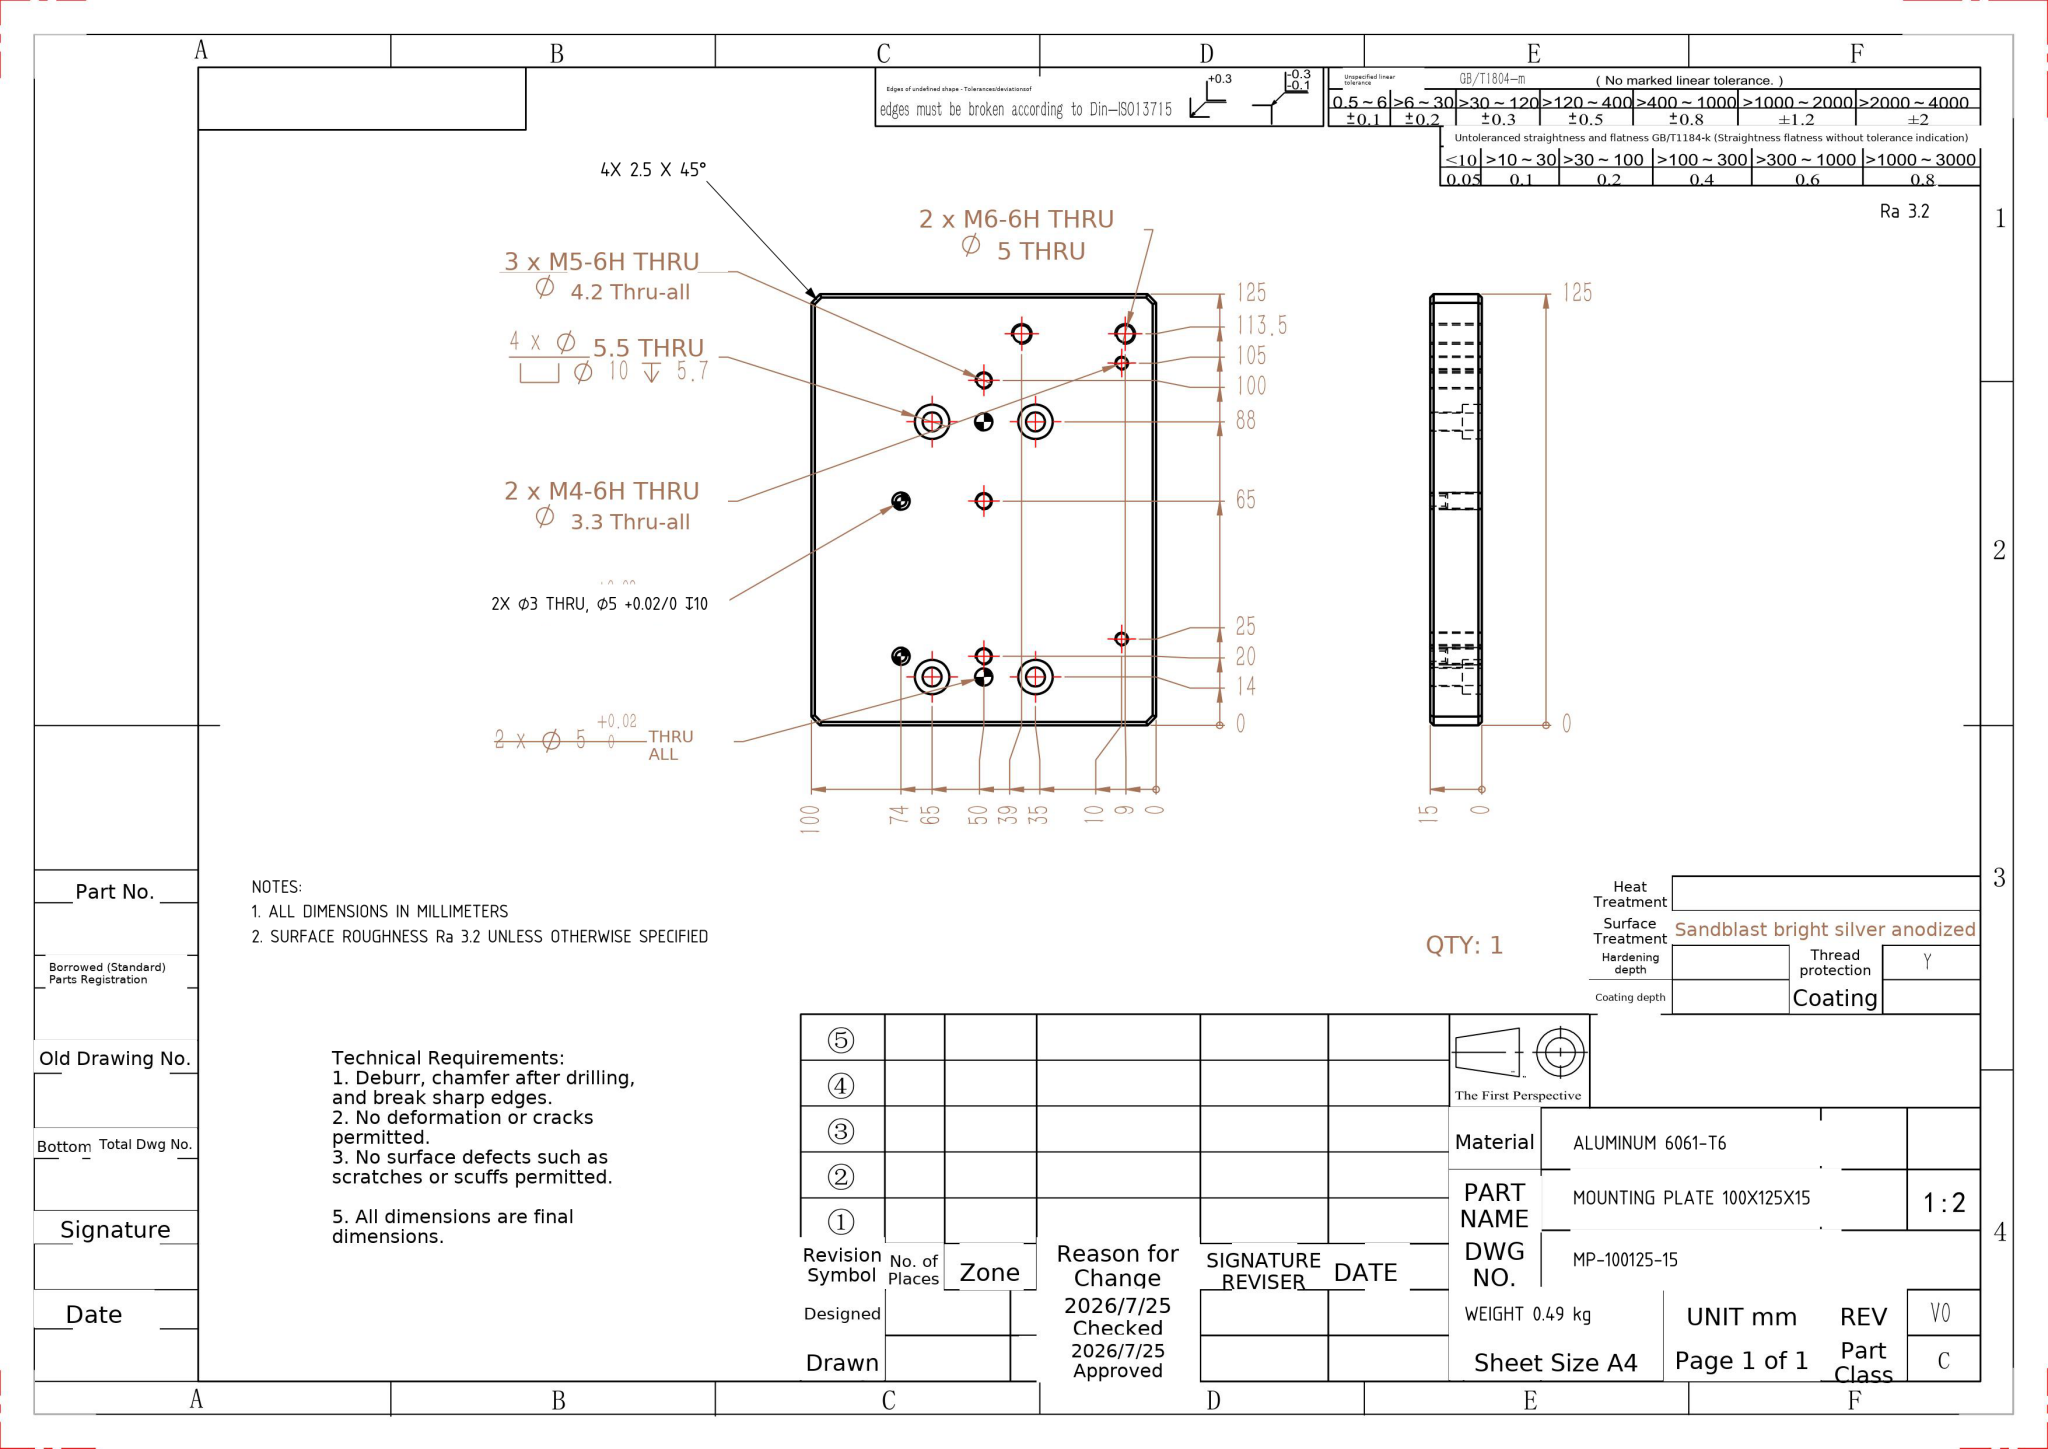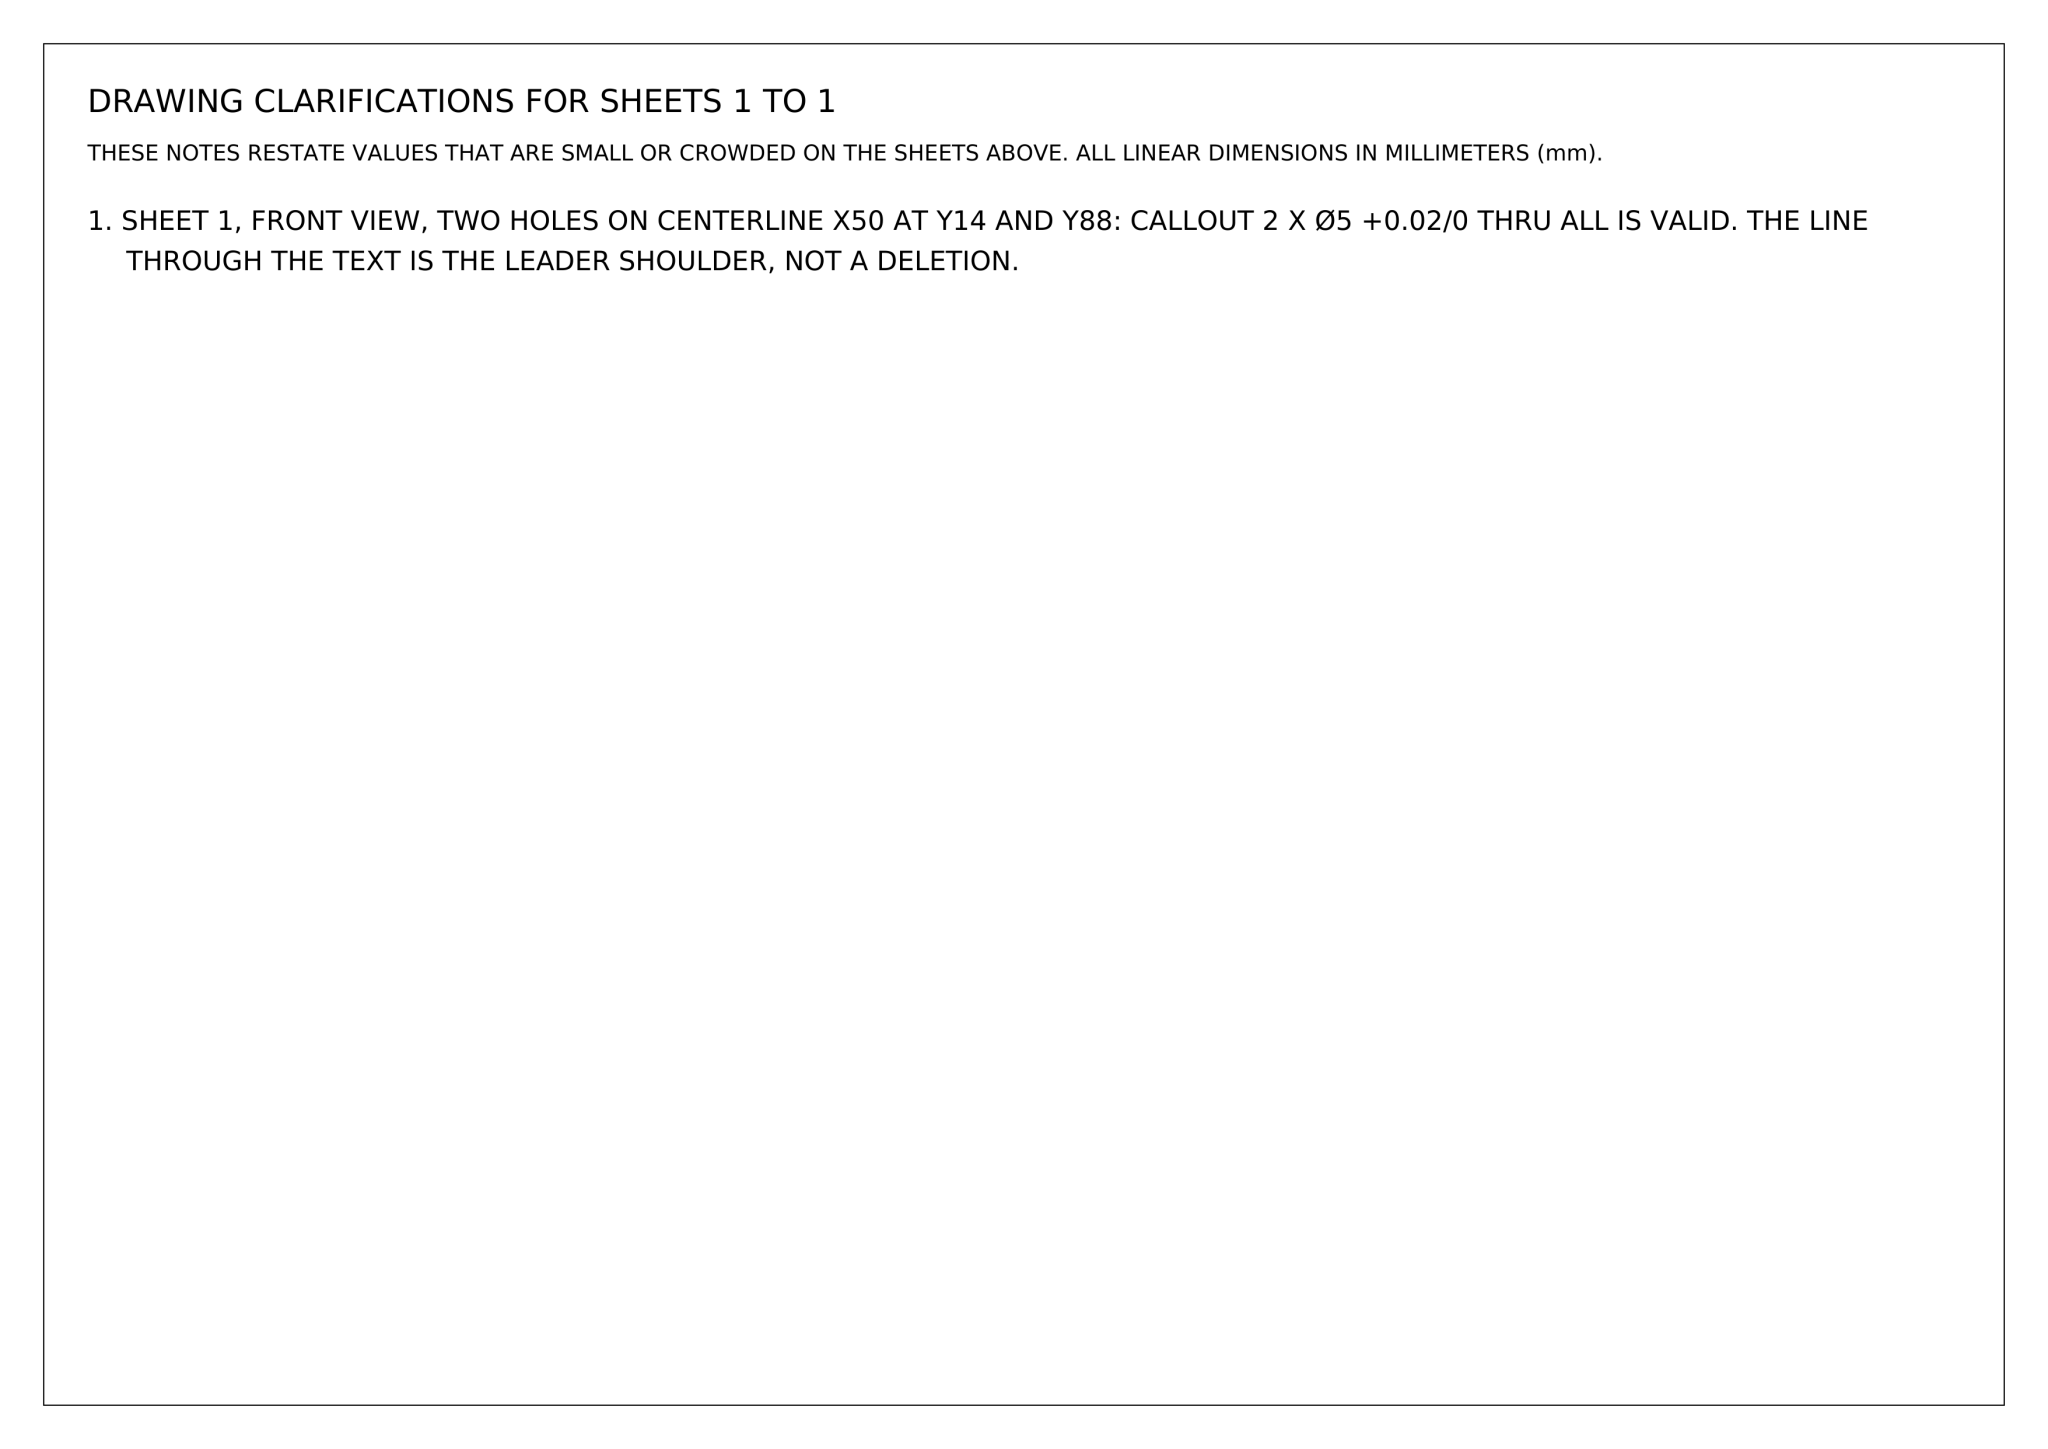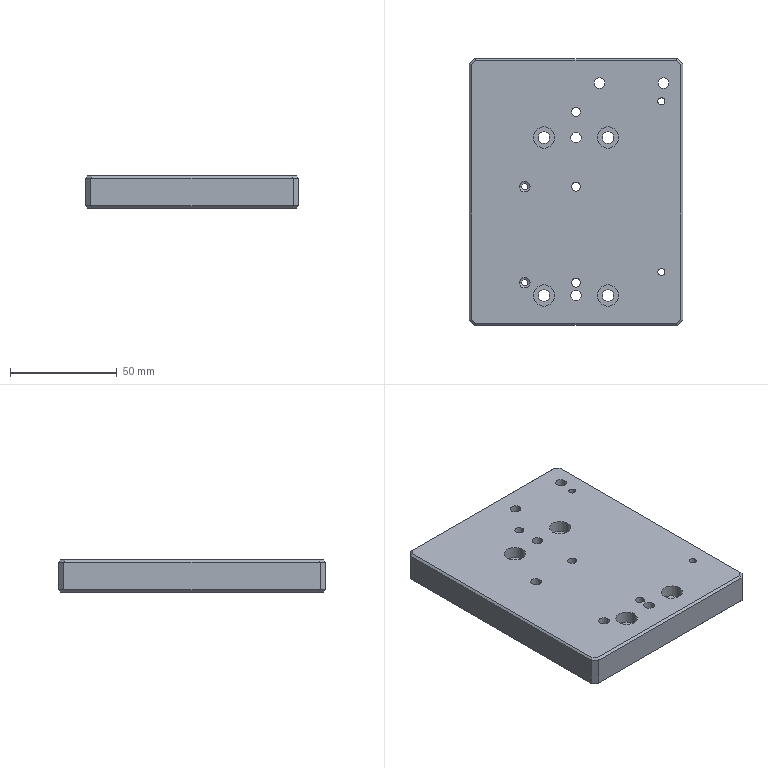Part | NX | mm | 1 solid | 76 faces | box 100 x 125 x 15 mm | volume 181668 mm3 | cylinder 42 | plane 30 | cone 4 | commonest cylinder face diameters 5 x12 10 x8 5.5 x8 4.2 x6 3.3 x4 3 x4